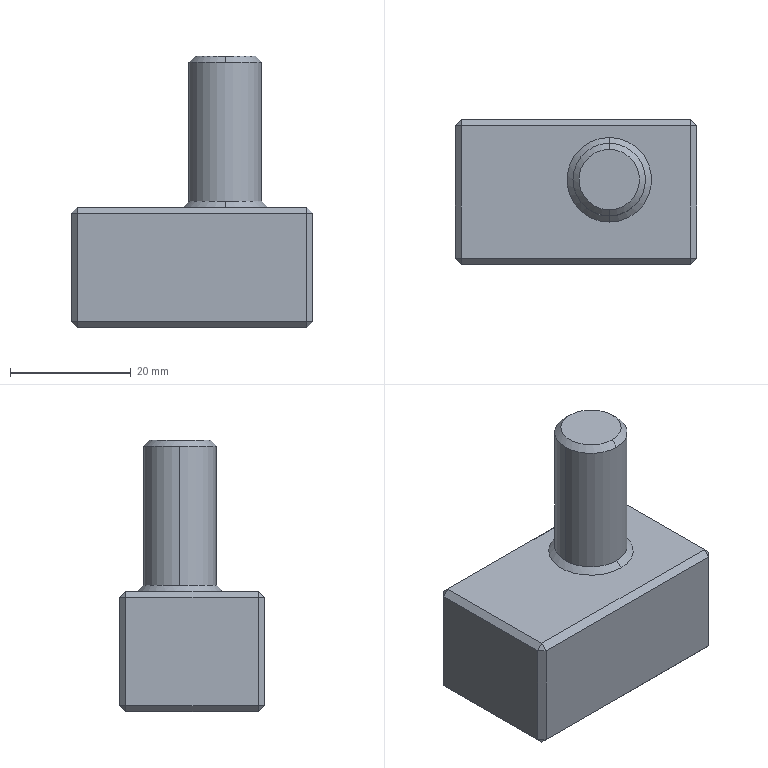Component | SolidWorks | LocatingPinB-1 | 1 solid | 33 faces | box 40 x 24 x 45 mm | volume 21867 mm3 | plane 27 | cone 4 | cylinder 2 | commonest cylinder face diameters 12 x2 | material Aviation Aluminum-7075
build123d program:
from build123d import *

# Parameters (mm, degrees)
SKETCH1_W           = 40
SKETCH1_H           = 20
BOSS_EXTRUDE1_DEPTH = 24
SKETCH2_R           = 6
BOSS_EXTRUDE2_DEPTH = 25
CHAMFER1_SIZE       = 1


with BuildPart() as part:
    # Sketch1 → Boss-Extrude1 (new body)
    with BuildSketch(Plane.XY):
        Rectangle(SKETCH1_W, SKETCH1_H)
    extrude(amount=BOSS_EXTRUDE1_DEPTH)

    # Sketch2 → Boss-Extrude2 (add)
    with BuildSketch(Plane.XZ.offset(10)):
        with Locations(Location((5.5, 14, 0), (0, 0, 180))):
            Circle(SKETCH2_R)
    extrude(amount=BOSS_EXTRUDE2_DEPTH)

    # Chamfer1
    chamfer1_edges = [part.edges().sort_by_distance(p)[0] for p in [
        (20, 0, 24),
        (0, 10, 24),
        (11.5, -10, 14),
        (11.5, -35, 14),
        (-20, 0, 24),
        (0, 10, 0),
        (20, 0, 0),
        (0, -10, 0),
        (-20, 0, 0),
        (0, -10, 24),
        (-20, 10, 12),
        (20, 10, 12),
        (20, -10, 12),
        (-20, -10, 12),
    ]]
    chamfer(chamfer1_edges, length=CHAMFER1_SIZE)


solid = part.part

# Placed as in the assembly
solid = solid.moved(Location((85.13, -406.626, 682.215), (-90, 0, 0)))
STEP:
#1=CARTESIAN_POINT('',(3.568,-15.655,28.237));
#2=VERTEX_POINT('',#1);
#3=CARTESIAN_POINT('',(3.568,-15.261,28.237));
#4=VERTEX_POINT('',#3);
#5=CARTESIAN_POINT('',(3.568,-15.458,28.237));
#6=DIRECTION('',(0.,-0.,1.));
#7=DIRECTION('',(1.,0.,0.));
#8=AXIS2_PLACEMENT_3D('',#5,#6,#7);
#9=CIRCLE('',#8,0.1969);
#10=EDGE_CURVE('',#2,#4,#9,.T.);
#11=ORIENTED_EDGE('',*,*,#10,.F.);
#12=CARTESIAN_POINT('',(3.568,-15.694,28.197));
#13=VERTEX_POINT('',#12);
#14=CARTESIAN_POINT('',(3.568,-15.655,28.237));
#15=DIRECTION('',(-0.,-0.7071,-0.7071));
#16=VECTOR('',#15,39.37);
#17=LINE('',#14,#16);
#18=EDGE_CURVE('',#2,#13,#17,.T.);
#19=ORIENTED_EDGE('',*,*,#18,.T.);
#20=CARTESIAN_POINT('',(3.804,-15.458,28.197));
#21=VERTEX_POINT('',#20);
#22=CARTESIAN_POINT('',(3.568,-15.458,28.197));
#23=DIRECTION('',(-0.,0.,-1.));
#24=DIRECTION('',(0.,-1.,0.));
#25=AXIS2_PLACEMENT_3D('',#22,#23,#24);
#26=CIRCLE('',#25,0.2362);
#27=EDGE_CURVE('',#21,#13,#26,.T.);
#28=ORIENTED_EDGE('',*,*,#27,.F.);
#29=CARTESIAN_POINT('',(3.568,-15.222,28.197));
#30=VERTEX_POINT('',#29);
#31=CARTESIAN_POINT('',(3.568,-15.458,28.197));
#32=DIRECTION('',(-0.,0.,-1.));
#33=DIRECTION('',(0.,-1.,0.));
#34=AXIS2_PLACEMENT_3D('',#31,#32,#33);
#35=CIRCLE('',#34,0.2362);
#36=EDGE_CURVE('',#30,#21,#35,.T.);
#37=ORIENTED_EDGE('',*,*,#36,.F.);
#38=CARTESIAN_POINT('',(3.568,-15.261,28.237));
#39=DIRECTION('',(-0.,0.7071,-0.7071));
#40=VECTOR('',#39,39.37);
#41=LINE('',#38,#40);
#42=EDGE_CURVE('',#4,#30,#41,.T.);
#43=ORIENTED_EDGE('',*,*,#42,.F.);
#44=EDGE_LOOP('',(#11,#19,#28,#37,#43));
#45=FACE_OUTER_BOUND('',#44,.T.);
#46=CARTESIAN_POINT('',(3.568,-15.458,28.237));
#47=DIRECTION('',(-0.,0.,-1.));
#48=DIRECTION('',(0.,1.,0.));
#49=AXIS2_PLACEMENT_3D('',#46,#47,#48);
#50=CONICAL_SURFACE('',#49,0.1969,0.7854);
#51=ADVANCED_FACE('',(#45),#50,.T.);
#52=CARTESIAN_POINT('',(3.568,-15.694,27.292));
#53=VERTEX_POINT('',#52);
#54=CARTESIAN_POINT('',(3.804,-15.458,27.292));
#55=VERTEX_POINT('',#54);
#56=CARTESIAN_POINT('',(3.568,-15.458,27.292));
#57=DIRECTION('',(0.,-0.,1.));
#58=DIRECTION('',(0.,1.,0.));
#59=AXIS2_PLACEMENT_3D('',#56,#57,#58);
#60=CIRCLE('',#59,0.2362);
#61=EDGE_CURVE('',#53,#55,#60,.T.);
#62=ORIENTED_EDGE('',*,*,#61,.F.);
#63=CARTESIAN_POINT('',(3.568,-15.733,27.253));
#64=VERTEX_POINT('',#63);
#65=CARTESIAN_POINT('',(3.568,-15.694,27.292));
#66=DIRECTION('',(-0.,-0.7071,-0.7071));
#67=VECTOR('',#66,39.37);
#68=LINE('',#65,#67);
#69=EDGE_CURVE('',#53,#64,#68,.T.);
#70=ORIENTED_EDGE('',*,*,#69,.T.);
#71=CARTESIAN_POINT('',(3.568,-15.182,27.253));
#72=VERTEX_POINT('',#71);
#73=CARTESIAN_POINT('',(3.568,-15.458,27.253));
#74=DIRECTION('',(-0.,0.,-1.));
#75=DIRECTION('',(-1.,0.,0.));
#76=AXIS2_PLACEMENT_3D('',#73,#74,#75);
#77=CIRCLE('',#76,0.2756);
#78=EDGE_CURVE('',#72,#64,#77,.T.);
#79=ORIENTED_EDGE('',*,*,#78,.F.);
#80=CARTESIAN_POINT('',(3.568,-15.222,27.292));
#81=VERTEX_POINT('',#80);
#82=CARTESIAN_POINT('',(3.568,-15.222,27.292));
#83=DIRECTION('',(-0.,0.7071,-0.7071));
#84=VECTOR('',#83,39.37);
#85=LINE('',#82,#84);
#86=EDGE_CURVE('',#81,#72,#85,.T.);
#87=ORIENTED_EDGE('',*,*,#86,.F.);
#88=CARTESIAN_POINT('',(3.568,-15.458,27.292));
#89=DIRECTION('',(0.,-0.,1.));
#90=DIRECTION('',(0.,1.,0.));
#91=AXIS2_PLACEMENT_3D('',#88,#89,#90);
#92=CIRCLE('',#91,0.2362);
#93=EDGE_CURVE('',#55,#81,#92,.T.);
#94=ORIENTED_EDGE('',*,*,#93,.F.);
#95=EDGE_LOOP('',(#62,#70,#79,#87,#94));
#96=FACE_OUTER_BOUND('',#95,.T.);
#97=CARTESIAN_POINT('',(3.568,-15.458,27.292));
#98=DIRECTION('',(-0.,0.,-1.));
#99=DIRECTION('',(0.,1.,0.));
#100=AXIS2_PLACEMENT_3D('',#97,#98,#99);
#101=CONICAL_SURFACE('',#100,0.2362,0.7854);
#102=ADVANCED_FACE('',(#96),#101,.T.);
#103=CARTESIAN_POINT('',(3.332,-15.458,28.197));
#104=VERTEX_POINT('',#103);
#105=CARTESIAN_POINT('',(3.568,-15.458,28.197));
#106=DIRECTION('',(-0.,0.,-1.));
#107=DIRECTION('',(0.,-1.,0.));
#108=AXIS2_PLACEMENT_3D('',#105,#106,#107);
#109=CIRCLE('',#108,0.2362);
#110=EDGE_CURVE('',#104,#30,#109,.T.);
#111=ORIENTED_EDGE('',*,*,#110,.T.);
#112=ORIENTED_EDGE('',*,*,#36,.T.);
#113=CARTESIAN_POINT('',(3.804,-15.458,28.237));
#114=DIRECTION('',(-0.,0.,-1.));
#115=VECTOR('',#114,39.37);
#116=LINE('',#113,#115);
#117=EDGE_CURVE('',#21,#55,#116,.T.);
#118=ORIENTED_EDGE('',*,*,#117,.T.);
#119=ORIENTED_EDGE('',*,*,#93,.T.);
#120=CARTESIAN_POINT('',(3.332,-15.458,27.292));
#121=VERTEX_POINT('',#120);
#122=CARTESIAN_POINT('',(3.568,-15.458,27.292));
#123=DIRECTION('',(0.,-0.,1.));
#124=DIRECTION('',(0.,1.,0.));
#125=AXIS2_PLACEMENT_3D('',#122,#123,#124);
#126=CIRCLE('',#125,0.2362);
#127=EDGE_CURVE('',#81,#121,#126,.T.);
#128=ORIENTED_EDGE('',*,*,#127,.T.);
#129=CARTESIAN_POINT('',(3.332,-15.458,28.237));
#130=DIRECTION('',(-0.,0.,-1.));
#131=VECTOR('',#130,39.37);
#132=LINE('',#129,#131);
#133=EDGE_CURVE('',#104,#121,#132,.T.);
#134=ORIENTED_EDGE('',*,*,#133,.F.);
#135=EDGE_LOOP('',(#111,#112,#118,#119,#128,#134));
#136=FACE_OUTER_BOUND('',#135,.T.);
#137=CARTESIAN_POINT('',(3.568,-15.458,28.237));
#138=DIRECTION('',(-0.,0.,-1.));
#139=DIRECTION('',(-1.,0.,0.));
#140=AXIS2_PLACEMENT_3D('',#137,#138,#139);
#141=CYLINDRICAL_SURFACE('',#140,0.2362);
#142=ADVANCED_FACE('',(#136),#141,.T.);
#143=ORIENTED_EDGE('',*,*,#78,.T.);
#144=CARTESIAN_POINT('',(3.568,-15.458,27.253));
#145=DIRECTION('',(-0.,0.,-1.));
#146=DIRECTION('',(-1.,0.,0.));
#147=AXIS2_PLACEMENT_3D('',#144,#145,#146);
#148=CIRCLE('',#147,0.2756);
#149=EDGE_CURVE('',#64,#72,#148,.T.);
#150=ORIENTED_EDGE('',*,*,#149,.T.);
#151=EDGE_LOOP('',(#143,#150));
#152=FACE_BOUND('',#151,.T.);
#153=CARTESIAN_POINT('',(2.604,-15.97,27.253));
#154=VERTEX_POINT('',#153);
#155=CARTESIAN_POINT('',(4.1,-15.97,27.253));
#156=VERTEX_POINT('',#155);
#157=CARTESIAN_POINT('',(4.139,-15.97,27.253));
#158=DIRECTION('',(1.,-0.,-0.));
#159=VECTOR('',#158,39.37);
#160=LINE('',#157,#159);
#161=EDGE_CURVE('',#154,#156,#160,.T.);
#162=ORIENTED_EDGE('',*,*,#161,.T.);
#163=CARTESIAN_POINT('',(4.1,-15.103,27.253));
#164=VERTEX_POINT('',#163);
#165=CARTESIAN_POINT('',(4.1,-15.064,27.253));
#166=DIRECTION('',(0.,1.,0.));
#167=VECTOR('',#166,39.37);
#168=LINE('',#165,#167);
#169=EDGE_CURVE('',#156,#164,#168,.T.);
#170=ORIENTED_EDGE('',*,*,#169,.T.);
#171=CARTESIAN_POINT('',(2.604,-15.103,27.253));
#172=VERTEX_POINT('',#171);
#173=CARTESIAN_POINT('',(2.564,-15.103,27.253));
#174=DIRECTION('',(-1.,0.,0.));
#175=VECTOR('',#174,39.37);
#176=LINE('',#173,#175);
#177=EDGE_CURVE('',#164,#172,#176,.T.);
#178=ORIENTED_EDGE('',*,*,#177,.T.);
#179=CARTESIAN_POINT('',(2.604,-15.064,27.253));
#180=DIRECTION('',(-0.,-1.,-0.));
#181=VECTOR('',#180,39.37);
#182=LINE('',#179,#181);
#183=EDGE_CURVE('',#172,#154,#182,.T.);
#184=ORIENTED_EDGE('',*,*,#183,.T.);
#185=EDGE_LOOP('',(#162,#170,#178,#184));
#186=FACE_OUTER_BOUND('',#185,.T.);
#187=CARTESIAN_POINT('',(4.139,-15.064,27.253));
#188=DIRECTION('',(-0.,0.,-1.));
#189=DIRECTION('',(-1.,0.,0.));
#190=AXIS2_PLACEMENT_3D('',#187,#188,#189);
#191=PLANE('',#190);
#192=ADVANCED_FACE('',(#152,#186),#191,.F.);
#193=CARTESIAN_POINT('',(2.564,-15.97,26.505));
#194=VERTEX_POINT('',#193);
#195=CARTESIAN_POINT('',(2.564,-15.97,27.213));
#196=VERTEX_POINT('',#195);
#197=CARTESIAN_POINT('',(2.564,-15.97,27.253));
#198=DIRECTION('',(0.,-0.,1.));
#199=VECTOR('',#198,39.37);
#200=LINE('',#197,#199);
#201=EDGE_CURVE('',#194,#196,#200,.T.);
#202=ORIENTED_EDGE('',*,*,#201,.T.);
#203=CARTESIAN_POINT('',(2.564,-15.103,27.213));
#204=VERTEX_POINT('',#203);
#205=CARTESIAN_POINT('',(2.564,-15.064,27.213));
#206=DIRECTION('',(0.,1.,0.));
#207=VECTOR('',#206,39.37);
#208=LINE('',#205,#207);
#209=EDGE_CURVE('',#196,#204,#208,.T.);
#210=ORIENTED_EDGE('',*,*,#209,.T.);
#211=CARTESIAN_POINT('',(2.564,-15.103,26.505));
#212=VERTEX_POINT('',#211);
#213=CARTESIAN_POINT('',(2.564,-15.103,26.465));
#214=DIRECTION('',(-0.,0.,-1.));
#215=VECTOR('',#214,39.37);
#216=LINE('',#213,#215);
#217=EDGE_CURVE('',#204,#212,#216,.T.);
#218=ORIENTED_EDGE('',*,*,#217,.T.);
#219=CARTESIAN_POINT('',(2.564,-15.064,26.505));
#220=DIRECTION('',(-0.,-1.,-0.));
#221=VECTOR('',#220,39.37);
#222=LINE('',#219,#221);
#223=EDGE_CURVE('',#212,#194,#222,.T.);
#224=ORIENTED_EDGE('',*,*,#223,.T.);
#225=EDGE_LOOP('',(#202,#210,#218,#224));
#226=FACE_OUTER_BOUND('',#225,.T.);
#227=CARTESIAN_POINT('',(2.564,-15.064,27.253));
#228=DIRECTION('',(1.,-0.,-0.));
#229=DIRECTION('',(-0.,0.,-1.));
#230=AXIS2_PLACEMENT_3D('',#227,#228,#229);
#231=PLANE('',#230);
#232=ADVANCED_FACE('',(#226),#231,.F.);
#233=CARTESIAN_POINT('',(4.139,-15.103,26.505));
#234=VERTEX_POINT('',#233);
#235=CARTESIAN_POINT('',(4.139,-15.103,27.213));
#236=VERTEX_POINT('',#235);
#237=CARTESIAN_POINT('',(4.139,-15.103,27.253));
#238=DIRECTION('',(0.,-0.,1.));
#239=VECTOR('',#238,39.37);
#240=LINE('',#237,#239);
#241=EDGE_CURVE('',#234,#236,#240,.T.);
#242=ORIENTED_EDGE('',*,*,#241,.T.);
#243=CARTESIAN_POINT('',(4.139,-15.97,27.213));
#244=VERTEX_POINT('',#243);
#245=CARTESIAN_POINT('',(4.139,-15.064,27.213));
#246=DIRECTION('',(-0.,-1.,-0.));
#247=VECTOR('',#246,39.37);
#248=LINE('',#245,#247);
#249=EDGE_CURVE('',#236,#244,#248,.T.);
#250=ORIENTED_EDGE('',*,*,#249,.T.);
#251=CARTESIAN_POINT('',(4.139,-15.97,26.505));
#252=VERTEX_POINT('',#251);
#253=CARTESIAN_POINT('',(4.139,-15.97,27.253));
#254=DIRECTION('',(-0.,0.,-1.));
#255=VECTOR('',#254,39.37);
#256=LINE('',#253,#255);
#257=EDGE_CURVE('',#244,#252,#256,.T.);
#258=ORIENTED_EDGE('',*,*,#257,.T.);
#259=CARTESIAN_POINT('',(4.139,-15.064,26.505));
#260=DIRECTION('',(0.,1.,0.));
#261=VECTOR('',#260,39.37);
#262=LINE('',#259,#261);
#263=EDGE_CURVE('',#252,#234,#262,.T.);
#264=ORIENTED_EDGE('',*,*,#263,.T.);
#265=EDGE_LOOP('',(#242,#250,#258,#264));
#266=FACE_OUTER_BOUND('',#265,.T.);
#267=CARTESIAN_POINT('',(4.139,-15.064,27.253));
#268=DIRECTION('',(-1.,0.,0.));
#269=DIRECTION('',(0.,1.,0.));
#270=AXIS2_PLACEMENT_3D('',#267,#268,#269);
#271=PLANE('',#270);
#272=ADVANCED_FACE('',(#266),#271,.F.);
#273=CARTESIAN_POINT('',(2.604,-15.103,26.465));
#274=VERTEX_POINT('',#273);
#275=CARTESIAN_POINT('',(4.1,-15.103,26.465));
#276=VERTEX_POINT('',#275);
#277=CARTESIAN_POINT('',(4.139,-15.103,26.465));
#278=DIRECTION('',(1.,-0.,-0.));
#279=VECTOR('',#278,39.37);
#280=LINE('',#277,#279);
#281=EDGE_CURVE('',#274,#276,#280,.T.);
#282=ORIENTED_EDGE('',*,*,#281,.T.);
#283=CARTESIAN_POINT('',(4.1,-15.97,26.465));
#284=VERTEX_POINT('',#283);
#285=CARTESIAN_POINT('',(4.1,-15.064,26.465));
#286=DIRECTION('',(-0.,-1.,-0.));
#287=VECTOR('',#286,39.37);
#288=LINE('',#285,#287);
#289=EDGE_CURVE('',#276,#284,#288,.T.);
#290=ORIENTED_EDGE('',*,*,#289,.T.);
#291=CARTESIAN_POINT('',(2.604,-15.97,26.465));
#292=VERTEX_POINT('',#291);
#293=CARTESIAN_POINT('',(4.139,-15.97,26.465));
#294=DIRECTION('',(-1.,0.,0.));
#295=VECTOR('',#294,39.37);
#296=LINE('',#293,#295);
#297=EDGE_CURVE('',#284,#292,#296,.T.);
#298=ORIENTED_EDGE('',*,*,#297,.T.);
#299=CARTESIAN_POINT('',(2.604,-15.064,26.465));
#300=DIRECTION('',(0.,1.,0.));
#301=VECTOR('',#300,39.37);
#302=LINE('',#299,#301);
#303=EDGE_CURVE('',#292,#274,#302,.T.);
#304=ORIENTED_EDGE('',*,*,#303,.T.);
#305=EDGE_LOOP('',(#282,#290,#298,#304));
#306=FACE_OUTER_BOUND('',#305,.T.);
#307=CARTESIAN_POINT('',(4.139,-15.064,26.465));
#308=DIRECTION('',(0.,-0.,1.));
#309=DIRECTION('',(1.,-0.,-0.));
#310=AXIS2_PLACEMENT_3D('',#307,#308,#309);
#311=PLANE('',#310);
#312=ADVANCED_FACE('',(#306),#311,.F.);
#313=CARTESIAN_POINT('',(2.604,-15.064,27.213));
#314=VERTEX_POINT('',#313);
#315=CARTESIAN_POINT('',(4.1,-15.064,27.213));
#316=VERTEX_POINT('',#315);
#317=CARTESIAN_POINT('',(4.139,-15.064,27.213));
#318=DIRECTION('',(1.,-0.,-0.));
#319=VECTOR('',#318,39.37);
#320=LINE('',#317,#319);
#321=EDGE_CURVE('',#314,#316,#320,.T.);
#322=ORIENTED_EDGE('',*,*,#321,.T.);
#323=CARTESIAN_POINT('',(4.1,-15.064,26.505));
#324=VERTEX_POINT('',#323);
#325=CARTESIAN_POINT('',(4.1,-15.064,26.465));
#326=DIRECTION('',(-0.,0.,-1.));
#327=VECTOR('',#326,39.37);
#328=LINE('',#325,#327);
#329=EDGE_CURVE('',#316,#324,#328,.T.);
#330=ORIENTED_EDGE('',*,*,#329,.T.);
#331=CARTESIAN_POINT('',(2.604,-15.064,26.505));
#332=VERTEX_POINT('',#331);
#333=CARTESIAN_POINT('',(2.564,-15.064,26.505));
#334=DIRECTION('',(-1.,0.,0.));
#335=VECTOR('',#334,39.37);
#336=LINE('',#333,#335);
#337=EDGE_CURVE('',#324,#332,#336,.T.);
#338=ORIENTED_EDGE('',*,*,#337,.T.);
#339=CARTESIAN_POINT('',(2.604,-15.064,27.253));
#340=DIRECTION('',(0.,-0.,1.));
#341=VECTOR('',#340,39.37);
#342=LINE('',#339,#341);
#343=EDGE_CURVE('',#332,#314,#342,.T.);
#344=ORIENTED_EDGE('',*,*,#343,.T.);
#345=EDGE_LOOP('',(#322,#330,#338,#344));
#346=FACE_OUTER_BOUND('',#345,.T.);
#347=CARTESIAN_POINT('',(3.352,-15.064,26.859));
#348=DIRECTION('',(0.,1.,0.));
#349=DIRECTION('',(1.,-0.,-0.));
#350=AXIS2_PLACEMENT_3D('',#347,#348,#349);
#351=PLANE('',#350);
#352=ADVANCED_FACE('',(#346),#351,.T.);
#353=CARTESIAN_POINT('',(4.1,-16.009,26.505));
#354=VERTEX_POINT('',#353);
#355=CARTESIAN_POINT('',(4.1,-16.009,27.213));
#356=VERTEX_POINT('',#355);
#357=CARTESIAN_POINT('',(4.1,-16.009,26.859));
#358=DIRECTION('',(0.,-0.,1.));
#359=VECTOR('',#358,39.37);
#360=LINE('',#357,#359);
#361=EDGE_CURVE('',#354,#356,#360,.T.);
#362=ORIENTED_EDGE('',*,*,#361,.T.);
#363=CARTESIAN_POINT('',(2.604,-16.009,27.213));
#364=VERTEX_POINT('',#363);
#365=CARTESIAN_POINT('',(3.352,-16.009,27.213));
#366=DIRECTION('',(-1.,0.,0.));
#367=VECTOR('',#366,39.37);
#368=LINE('',#365,#367);
#369=EDGE_CURVE('',#356,#364,#368,.T.);
#370=ORIENTED_EDGE('',*,*,#369,.T.);
#371=CARTESIAN_POINT('',(2.604,-16.009,26.505));
#372=VERTEX_POINT('',#371);
#373=CARTESIAN_POINT('',(2.604,-16.009,26.859));
#374=DIRECTION('',(-0.,0.,-1.));
#375=VECTOR('',#374,39.37);
#376=LINE('',#373,#375);
#377=EDGE_CURVE('',#364,#372,#376,.T.);
#378=ORIENTED_EDGE('',*,*,#377,.T.);
#379=CARTESIAN_POINT('',(3.352,-16.009,26.505));
#380=DIRECTION('',(1.,-0.,-0.));
#381=VECTOR('',#380,39.37);
#382=LINE('',#379,#381);
#383=EDGE_CURVE('',#372,#354,#382,.T.);
#384=ORIENTED_EDGE('',*,*,#383,.T.);
#385=EDGE_LOOP('',(#362,#370,#378,#384));
#386=FACE_OUTER_BOUND('',#385,.T.);
#387=CARTESIAN_POINT('',(3.352,-16.009,26.859));
#388=DIRECTION('',(0.,1.,0.));
#389=DIRECTION('',(1.,-0.,-0.));
#390=AXIS2_PLACEMENT_3D('',#387,#388,#389);
#391=PLANE('',#390);
#392=ADVANCED_FACE('',(#386),#391,.F.);
#393=ORIENTED_EDGE('',*,*,#117,.F.);
#394=ORIENTED_EDGE('',*,*,#27,.T.);
#395=CARTESIAN_POINT('',(3.568,-15.458,28.197));
#396=DIRECTION('',(-0.,0.,-1.));
#397=DIRECTION('',(0.,-1.,0.));
#398=AXIS2_PLACEMENT_3D('',#395,#396,#397);
#399=CIRCLE('',#398,0.2362);
#400=EDGE_CURVE('',#13,#104,#399,.T.);
#401=ORIENTED_EDGE('',*,*,#400,.T.);
#402=ORIENTED_EDGE('',*,*,#133,.T.);
#403=CARTESIAN_POINT('',(3.568,-15.458,27.292));
#404=DIRECTION('',(0.,-0.,1.));
#405=DIRECTION('',(0.,1.,0.));
#406=AXIS2_PLACEMENT_3D('',#403,#404,#405);
#407=CIRCLE('',#406,0.2362);
#408=EDGE_CURVE('',#121,#53,#407,.T.);
#409=ORIENTED_EDGE('',*,*,#408,.T.);
#410=ORIENTED_EDGE('',*,*,#61,.T.);
#411=EDGE_LOOP('',(#393,#394,#401,#402,#409,#410));
#412=FACE_OUTER_BOUND('',#411,.T.);
#413=CARTESIAN_POINT('',(3.568,-15.458,28.237));
#414=DIRECTION('',(-0.,0.,-1.));
#415=DIRECTION('',(-1.,0.,0.));
#416=AXIS2_PLACEMENT_3D('',#413,#414,#415);
#417=CYLINDRICAL_SURFACE('',#416,0.2362);
#418=ADVANCED_FACE('',(#412),#417,.T.);
#419=CARTESIAN_POINT('',(3.568,-15.458,28.237));
#420=DIRECTION('',(0.,-0.,1.));
#421=DIRECTION('',(1.,0.,0.));
#422=AXIS2_PLACEMENT_3D('',#419,#420,#421);
#423=CIRCLE('',#422,0.1969);
#424=EDGE_CURVE('',#4,#2,#423,.T.);
#425=ORIENTED_EDGE('',*,*,#424,.T.);
#426=ORIENTED_EDGE('',*,*,#10,.T.);
#427=EDGE_LOOP('',(#425,#426));
#428=FACE_OUTER_BOUND('',#427,.T.);
#429=CARTESIAN_POINT('',(3.568,-15.458,28.237));
#430=DIRECTION('',(0.,-0.,1.));
#431=DIRECTION('',(1.,-0.,-0.));
#432=AXIS2_PLACEMENT_3D('',#429,#430,#431);
#433=PLANE('',#432);
#434=ADVANCED_FACE('',(#428),#433,.T.);
#435=ORIENTED_EDGE('',*,*,#69,.F.);
#436=ORIENTED_EDGE('',*,*,#408,.F.);
#437=ORIENTED_EDGE('',*,*,#127,.F.);
#438=ORIENTED_EDGE('',*,*,#86,.T.);
#439=ORIENTED_EDGE('',*,*,#149,.F.);
#440=EDGE_LOOP('',(#435,#436,#437,#438,#439));
#441=FACE_OUTER_BOUND('',#440,.T.);
#442=CARTESIAN_POINT('',(3.568,-15.458,27.292));
#443=DIRECTION('',(-0.,0.,-1.));
#444=DIRECTION('',(0.,1.,0.));
#445=AXIS2_PLACEMENT_3D('',#442,#443,#444);
#446=CONICAL_SURFACE('',#445,0.2362,0.7854);
#447=ADVANCED_FACE('',(#441),#446,.T.);
#448=CARTESIAN_POINT('',(2.564,-15.103,26.505));
#449=DIRECTION('',(-0.7071,-0.,0.7071));
#450=VECTOR('',#449,39.37);
#451=LINE('',#448,#450);
#452=EDGE_CURVE('',#274,#212,#451,.T.);
#453=ORIENTED_EDGE('',*,*,#452,.F.);
#454=ORIENTED_EDGE('',*,*,#303,.F.);
#455=CARTESIAN_POINT('',(2.584,-15.97,26.485));
#456=DIRECTION('',(0.7071,-0.,-0.7071));
#457=VECTOR('',#456,39.37);
#458=LINE('',#455,#457);
#459=EDGE_CURVE('',#194,#292,#458,.T.);
#460=ORIENTED_EDGE('',*,*,#459,.F.);
#461=ORIENTED_EDGE('',*,*,#223,.F.);
#462=EDGE_LOOP('',(#453,#454,#460,#461));
#463=FACE_OUTER_BOUND('',#462,.T.);
#464=CARTESIAN_POINT('',(2.564,-15.064,26.505));
#465=DIRECTION('',(0.7071,-0.,0.7071));
#466=DIRECTION('',(-0.,-1.,-0.));
#467=AXIS2_PLACEMENT_3D('',#464,#465,#466);
#468=PLANE('',#467);
#469=ADVANCED_FACE('',(#463),#468,.F.);
#470=CARTESIAN_POINT('',(2.604,-15.084,26.485));
#471=DIRECTION('',(-0.,0.7071,0.7071));
#472=VECTOR('',#471,39.37);
#473=LINE('',#470,#472);
#474=EDGE_CURVE('',#274,#332,#473,.T.);
#475=ORIENTED_EDGE('',*,*,#474,.F.);
#476=ORIENTED_EDGE('',*,*,#452,.T.);
#477=CARTESIAN_POINT('',(2.564,-15.103,26.505));
#478=DIRECTION('',(-0.7071,-0.7071,0.));
#479=VECTOR('',#478,39.37);
#480=LINE('',#477,#479);
#481=EDGE_CURVE('',#332,#212,#480,.T.);
#482=ORIENTED_EDGE('',*,*,#481,.F.);
#483=EDGE_LOOP('',(#475,#476,#482));
#484=FACE_OUTER_BOUND('',#483,.T.);
#485=CARTESIAN_POINT('',(2.564,-15.103,26.505));
#486=DIRECTION('',(-0.5774,0.5774,-0.5774));
#487=DIRECTION('',(0.7071,0.7071,0.));
#488=AXIS2_PLACEMENT_3D('',#485,#486,#487);
#489=PLANE('',#488);
#490=ADVANCED_FACE('',(#484),#489,.T.);
#491=CARTESIAN_POINT('',(2.604,-16.009,26.505));
#492=DIRECTION('',(0.7071,-0.7071,0.));
#493=VECTOR('',#492,39.37);
#494=LINE('',#491,#493);
#495=EDGE_CURVE('',#194,#372,#494,.T.);
#496=ORIENTED_EDGE('',*,*,#495,.F.);
#497=ORIENTED_EDGE('',*,*,#459,.T.);
#498=CARTESIAN_POINT('',(2.604,-16.009,26.505));
#499=DIRECTION('',(-0.,0.7071,-0.7071));
#500=VECTOR('',#499,39.37);
#501=LINE('',#498,#500);
#502=EDGE_CURVE('',#372,#292,#501,.T.);
#503=ORIENTED_EDGE('',*,*,#502,.F.);
#504=EDGE_LOOP('',(#496,#497,#503));
#505=FACE_OUTER_BOUND('',#504,.T.);
#506=CARTESIAN_POINT('',(2.604,-16.009,26.505));
#507=DIRECTION('',(-0.5774,-0.5774,-0.5774));
#508=DIRECTION('',(-0.7071,0.7071,0.));
#509=AXIS2_PLACEMENT_3D('',#506,#507,#508);
#510=PLANE('',#509);
#511=ADVANCED_FACE('',(#505),#510,.T.);
#512=ORIENTED_EDGE('',*,*,#481,.T.);
#513=ORIENTED_EDGE('',*,*,#217,.F.);
#514=CARTESIAN_POINT('',(2.564,-15.103,27.213));
#515=DIRECTION('',(-0.7071,-0.7071,-0.));
#516=VECTOR('',#515,39.37);
#517=LINE('',#514,#516);
#518=EDGE_CURVE('',#314,#204,#517,.T.);
#519=ORIENTED_EDGE('',*,*,#518,.F.);
#520=ORIENTED_EDGE('',*,*,#343,.F.);
#521=EDGE_LOOP('',(#512,#513,#519,#520));
#522=FACE_OUTER_BOUND('',#521,.T.);
#523=CARTESIAN_POINT('',(2.604,-15.064,26.859));
#524=DIRECTION('',(-0.7071,0.7071,0.));
#525=DIRECTION('',(-0.,0.,-1.));
#526=AXIS2_PLACEMENT_3D('',#523,#524,#525);
#527=PLANE('',#526);
#528=ADVANCED_FACE('',(#522),#527,.T.);
#529=ORIENTED_EDGE('',*,*,#474,.T.);
#530=ORIENTED_EDGE('',*,*,#337,.F.);
#531=CARTESIAN_POINT('',(4.1,-15.064,26.505));
#532=DIRECTION('',(0.,0.7071,0.7071));
#533=VECTOR('',#532,39.37);
#534=LINE('',#531,#533);
#535=EDGE_CURVE('',#276,#324,#534,.T.);
#536=ORIENTED_EDGE('',*,*,#535,.F.);
#537=ORIENTED_EDGE('',*,*,#281,.F.);
#538=EDGE_LOOP('',(#529,#530,#536,#537));
#539=FACE_OUTER_BOUND('',#538,.T.);
#540=CARTESIAN_POINT('',(3.352,-15.064,26.505));
#541=DIRECTION('',(-0.,0.7071,-0.7071));
#542=DIRECTION('',(1.,-0.,-0.));
#543=AXIS2_PLACEMENT_3D('',#540,#541,#542);
#544=PLANE('',#543);
#545=ADVANCED_FACE('',(#539),#544,.T.);
#546=CARTESIAN_POINT('',(4.139,-15.97,26.505));
#547=DIRECTION('',(0.7071,-0.,0.7071));
#548=VECTOR('',#547,39.37);
#549=LINE('',#546,#548);
#550=EDGE_CURVE('',#284,#252,#549,.T.);
#551=ORIENTED_EDGE('',*,*,#550,.F.);
#552=ORIENTED_EDGE('',*,*,#289,.F.);
#553=CARTESIAN_POINT('',(4.119,-15.103,26.485));
#554=DIRECTION('',(-0.7071,0.,-0.7071));
#555=VECTOR('',#554,39.37);
#556=LINE('',#553,#555);
#557=EDGE_CURVE('',#234,#276,#556,.T.);
#558=ORIENTED_EDGE('',*,*,#557,.F.);
#559=ORIENTED_EDGE('',*,*,#263,.F.);
#560=EDGE_LOOP('',(#551,#552,#558,#559));
#561=FACE_OUTER_BOUND('',#560,.T.);
#562=CARTESIAN_POINT('',(4.1,-15.064,26.465));
#563=DIRECTION('',(-0.7071,-0.,0.7071));
#564=DIRECTION('',(-0.,-1.,-0.));
#565=AXIS2_PLACEMENT_3D('',#562,#563,#564);
#566=PLANE('',#565);
#567=ADVANCED_FACE('',(#561),#566,.F.);
#568=ORIENTED_EDGE('',*,*,#502,.T.);
#569=ORIENTED_EDGE('',*,*,#297,.F.);
#570=CARTESIAN_POINT('',(4.1,-15.989,26.485));
#571=DIRECTION('',(0.,0.7071,-0.7071));
#572=VECTOR('',#571,39.37);
#573=LINE('',#570,#572);
#574=EDGE_CURVE('',#354,#284,#573,.T.);
#575=ORIENTED_EDGE('',*,*,#574,.F.);
#576=ORIENTED_EDGE('',*,*,#383,.F.);
#577=EDGE_LOOP('',(#568,#569,#575,#576));
#578=FACE_OUTER_BOUND('',#577,.T.);
#579=CARTESIAN_POINT('',(4.139,-15.97,26.465));
#580=DIRECTION('',(0.,0.7071,0.7071));
#581=DIRECTION('',(-1.,0.,0.));
#582=AXIS2_PLACEMENT_3D('',#579,#580,#581);
#583=PLANE('',#582);
#584=ADVANCED_FACE('',(#578),#583,.F.);
#585=ORIENTED_EDGE('',*,*,#495,.T.);
#586=ORIENTED_EDGE('',*,*,#377,.F.);
#587=CARTESIAN_POINT('',(2.604,-16.009,27.213));
#588=DIRECTION('',(0.7071,-0.7071,-0.));
#589=VECTOR('',#588,39.37);
#590=LINE('',#587,#589);
#591=EDGE_CURVE('',#196,#364,#590,.T.);
#592=ORIENTED_EDGE('',*,*,#591,.F.);
#593=ORIENTED_EDGE('',*,*,#201,.F.);
#594=EDGE_LOOP('',(#585,#586,#592,#593));
#595=FACE_OUTER_BOUND('',#594,.T.);
#596=CARTESIAN_POINT('',(2.564,-15.97,27.253));
#597=DIRECTION('',(0.7071,0.7071,0.));
#598=DIRECTION('',(0.,-0.,1.));
#599=AXIS2_PLACEMENT_3D('',#596,#597,#598);
#600=PLANE('',#599);
#601=ADVANCED_FACE('',(#595),#600,.F.);
#602=CARTESIAN_POINT('',(2.564,-15.103,27.213));
#603=DIRECTION('',(0.7071,-0.,0.7071));
#604=VECTOR('',#603,39.37);
#605=LINE('',#602,#604);
#606=EDGE_CURVE('',#204,#172,#605,.T.);
#607=ORIENTED_EDGE('',*,*,#606,.F.);
#608=ORIENTED_EDGE('',*,*,#209,.F.);
#609=CARTESIAN_POINT('',(2.584,-15.97,27.233));
#610=DIRECTION('',(-0.7071,0.,-0.7071));
#611=VECTOR('',#610,39.37);
#612=LINE('',#609,#611);
#613=EDGE_CURVE('',#154,#196,#612,.T.);
#614=ORIENTED_EDGE('',*,*,#613,.F.);
#615=ORIENTED_EDGE('',*,*,#183,.F.);
#616=EDGE_LOOP('',(#607,#608,#614,#615));
#617=FACE_OUTER_BOUND('',#616,.T.);
#618=CARTESIAN_POINT('',(2.604,-15.064,27.253));
#619=DIRECTION('',(0.7071,0.,-0.7071));
#620=DIRECTION('',(-0.,-1.,-0.));
#621=AXIS2_PLACEMENT_3D('',#618,#619,#620);
#622=PLANE('',#621);
#623=ADVANCED_FACE('',(#617),#622,.F.);
#624=ORIENTED_EDGE('',*,*,#518,.T.);
#625=ORIENTED_EDGE('',*,*,#606,.T.);
#626=CARTESIAN_POINT('',(2.604,-15.084,27.233));
#627=DIRECTION('',(-0.,-0.7071,0.7071));
#628=VECTOR('',#627,39.37);
#629=LINE('',#626,#628);
#630=EDGE_CURVE('',#314,#172,#629,.T.);
#631=ORIENTED_EDGE('',*,*,#630,.F.);
#632=EDGE_LOOP('',(#624,#625,#631));
#633=FACE_OUTER_BOUND('',#632,.T.);
#634=CARTESIAN_POINT('',(2.564,-15.103,27.213));
#635=DIRECTION('',(-0.5774,0.5774,0.5774));
#636=DIRECTION('',(0.7071,-0.,0.7071));
#637=AXIS2_PLACEMENT_3D('',#634,#635,#636);
#638=PLANE('',#637);
#639=ADVANCED_FACE('',(#633),#638,.T.);
#640=ORIENTED_EDGE('',*,*,#557,.T.);
#641=ORIENTED_EDGE('',*,*,#535,.T.);
#642=CARTESIAN_POINT('',(4.1,-15.064,26.505));
#643=DIRECTION('',(-0.7071,0.7071,0.));
#644=VECTOR('',#643,39.37);
#645=LINE('',#642,#644);
#646=EDGE_CURVE('',#234,#324,#645,.T.);
#647=ORIENTED_EDGE('',*,*,#646,.F.);
#648=EDGE_LOOP('',(#640,#641,#647));
#649=FACE_OUTER_BOUND('',#648,.T.);
#650=CARTESIAN_POINT('',(4.1,-15.064,26.505));
#651=DIRECTION('',(0.5774,0.5774,-0.5774));
#652=DIRECTION('',(0.7071,-0.7071,-0.));
#653=AXIS2_PLACEMENT_3D('',#650,#651,#652);
#654=PLANE('',#653);
#655=ADVANCED_FACE('',(#649),#654,.T.);
#656=ORIENTED_EDGE('',*,*,#574,.T.);
#657=ORIENTED_EDGE('',*,*,#550,.T.);
#658=CARTESIAN_POINT('',(4.139,-15.97,26.505));
#659=DIRECTION('',(0.7071,0.7071,-0.));
#660=VECTOR('',#659,39.37);
#661=LINE('',#658,#660);
#662=EDGE_CURVE('',#354,#252,#661,.T.);
#663=ORIENTED_EDGE('',*,*,#662,.F.);
#664=EDGE_LOOP('',(#656,#657,#663));
#665=FACE_OUTER_BOUND('',#664,.T.);
#666=CARTESIAN_POINT('',(4.139,-15.97,26.505));
#667=DIRECTION('',(0.5774,-0.5774,-0.5774));
#668=DIRECTION('',(-0.7071,-0.7071,-0.));
#669=AXIS2_PLACEMENT_3D('',#666,#667,#668);
#670=PLANE('',#669);
#671=ADVANCED_FACE('',(#665),#670,.T.);
#672=ORIENTED_EDGE('',*,*,#613,.T.);
#673=ORIENTED_EDGE('',*,*,#591,.T.);
#674=CARTESIAN_POINT('',(2.604,-16.009,27.213));
#675=DIRECTION('',(0.,-0.7071,-0.7071));
#676=VECTOR('',#675,39.37);
#677=LINE('',#674,#676);
#678=EDGE_CURVE('',#154,#364,#677,.T.);
#679=ORIENTED_EDGE('',*,*,#678,.F.);
#680=EDGE_LOOP('',(#672,#673,#679));
#681=FACE_OUTER_BOUND('',#680,.T.);
#682=CARTESIAN_POINT('',(2.604,-16.009,27.213));
#683=DIRECTION('',(-0.5774,-0.5774,0.5774));
#684=DIRECTION('',(-0.7071,0.7071,0.));
#685=AXIS2_PLACEMENT_3D('',#682,#683,#684);
#686=PLANE('',#685);
#687=ADVANCED_FACE('',(#681),#686,.T.);
#688=ORIENTED_EDGE('',*,*,#630,.T.);
#689=ORIENTED_EDGE('',*,*,#177,.F.);
#690=CARTESIAN_POINT('',(4.1,-15.103,27.253));
#691=DIRECTION('',(-0.,-0.7071,0.7071));
#692=VECTOR('',#691,39.37);
#693=LINE('',#690,#692);
#694=EDGE_CURVE('',#316,#164,#693,.T.);
#695=ORIENTED_EDGE('',*,*,#694,.F.);
#696=ORIENTED_EDGE('',*,*,#321,.F.);
#697=EDGE_LOOP('',(#688,#689,#695,#696));
#698=FACE_OUTER_BOUND('',#697,.T.);
#699=CARTESIAN_POINT('',(3.352,-15.064,27.213));
#700=DIRECTION('',(0.,0.7071,0.7071));
#701=DIRECTION('',(-1.,0.,0.));
#702=AXIS2_PLACEMENT_3D('',#699,#700,#701);
#703=PLANE('',#702);
#704=ADVANCED_FACE('',(#698),#703,.T.);
#705=ORIENTED_EDGE('',*,*,#646,.T.);
#706=ORIENTED_EDGE('',*,*,#329,.F.);
#707=CARTESIAN_POINT('',(4.119,-15.084,27.213));
#708=DIRECTION('',(-0.7071,0.7071,0.));
#709=VECTOR('',#708,39.37);
#710=LINE('',#707,#709);
#711=EDGE_CURVE('',#236,#316,#710,.T.);
#712=ORIENTED_EDGE('',*,*,#711,.F.);
#713=ORIENTED_EDGE('',*,*,#241,.F.);
#714=EDGE_LOOP('',(#705,#706,#712,#713));
#715=FACE_OUTER_BOUND('',#714,.T.);
#716=CARTESIAN_POINT('',(4.1,-15.064,26.859));
#717=DIRECTION('',(0.7071,0.7071,0.));
#718=DIRECTION('',(0.,-0.,1.));
#719=AXIS2_PLACEMENT_3D('',#716,#717,#718);
#720=PLANE('',#719);
#721=ADVANCED_FACE('',(#715),#720,.T.);
#722=ORIENTED_EDGE('',*,*,#662,.T.);
#723=ORIENTED_EDGE('',*,*,#257,.F.);
#724=CARTESIAN_POINT('',(4.139,-15.97,27.213));
#725=DIRECTION('',(0.7071,0.7071,0.));
#726=VECTOR('',#725,39.37);
#727=LINE('',#724,#726);
#728=EDGE_CURVE('',#356,#244,#727,.T.);
#729=ORIENTED_EDGE('',*,*,#728,.F.);
#730=ORIENTED_EDGE('',*,*,#361,.F.);
#731=EDGE_LOOP('',(#722,#723,#729,#730));
#732=FACE_OUTER_BOUND('',#731,.T.);
#733=CARTESIAN_POINT('',(4.139,-15.97,27.253));
#734=DIRECTION('',(-0.7071,0.7071,0.));
#735=DIRECTION('',(-0.,0.,-1.));
#736=AXIS2_PLACEMENT_3D('',#733,#734,#735);
#737=PLANE('',#736);
#738=ADVANCED_FACE('',(#732),#737,.F.);
#739=ORIENTED_EDGE('',*,*,#678,.T.);
#740=ORIENTED_EDGE('',*,*,#369,.F.);
#741=CARTESIAN_POINT('',(4.1,-15.989,27.233));
#742=DIRECTION('',(-0.,-0.7071,-0.7071));
#743=VECTOR('',#742,39.37);
#744=LINE('',#741,#743);
#745=EDGE_CURVE('',#156,#356,#744,.T.);
#746=ORIENTED_EDGE('',*,*,#745,.F.);
#747=ORIENTED_EDGE('',*,*,#161,.F.);
#748=EDGE_LOOP('',(#739,#740,#746,#747));
#749=FACE_OUTER_BOUND('',#748,.T.);
#750=CARTESIAN_POINT('',(4.139,-15.97,27.253));
#751=DIRECTION('',(-0.,0.7071,-0.7071));
#752=DIRECTION('',(1.,-0.,-0.));
#753=AXIS2_PLACEMENT_3D('',#750,#751,#752);
#754=PLANE('',#753);
#755=ADVANCED_FACE('',(#749),#754,.F.);
#756=ORIENTED_EDGE('',*,*,#711,.T.);
#757=ORIENTED_EDGE('',*,*,#694,.T.);
#758=CARTESIAN_POINT('',(4.1,-15.103,27.253));
#759=DIRECTION('',(-0.7071,-0.,0.7071));
#760=VECTOR('',#759,39.37);
#761=LINE('',#758,#760);
#762=EDGE_CURVE('',#236,#164,#761,.T.);
#763=ORIENTED_EDGE('',*,*,#762,.F.);
#764=EDGE_LOOP('',(#756,#757,#763));
#765=FACE_OUTER_BOUND('',#764,.T.);
#766=CARTESIAN_POINT('',(4.1,-15.103,27.253));
#767=DIRECTION('',(0.5774,0.5774,0.5774));
#768=DIRECTION('',(0.7071,0.,-0.7071));
#769=AXIS2_PLACEMENT_3D('',#766,#767,#768);
#770=PLANE('',#769);
#771=ADVANCED_FACE('',(#765),#770,.T.);
#772=ORIENTED_EDGE('',*,*,#745,.T.);
#773=ORIENTED_EDGE('',*,*,#728,.T.);
#774=CARTESIAN_POINT('',(4.139,-15.97,27.213));
#775=DIRECTION('',(0.7071,0.,-0.7071));
#776=VECTOR('',#775,39.37);
#777=LINE('',#774,#776);
#778=EDGE_CURVE('',#156,#244,#777,.T.);
#779=ORIENTED_EDGE('',*,*,#778,.F.);
#780=EDGE_LOOP('',(#772,#773,#779));
#781=FACE_OUTER_BOUND('',#780,.T.);
#782=CARTESIAN_POINT('',(4.139,-15.97,27.213));
#783=DIRECTION('',(0.5774,-0.5774,0.5774));
#784=DIRECTION('',(-0.,-0.7071,-0.7071));
#785=AXIS2_PLACEMENT_3D('',#782,#783,#784);
#786=PLANE('',#785);
#787=ADVANCED_FACE('',(#781),#786,.T.);
#788=ORIENTED_EDGE('',*,*,#762,.T.);
#789=ORIENTED_EDGE('',*,*,#169,.F.);
#790=ORIENTED_EDGE('',*,*,#778,.T.);
#791=ORIENTED_EDGE('',*,*,#249,.F.);
#792=EDGE_LOOP('',(#788,#789,#790,#791));
#793=FACE_OUTER_BOUND('',#792,.T.);
#794=CARTESIAN_POINT('',(4.139,-15.064,27.213));
#795=DIRECTION('',(-0.7071,0.,-0.7071));
#796=DIRECTION('',(-0.,-1.,-0.));
#797=AXIS2_PLACEMENT_3D('',#794,#795,#796);
#798=PLANE('',#797);
#799=ADVANCED_FACE('',(#793),#798,.F.);
#800=ORIENTED_EDGE('',*,*,#18,.F.);
#801=ORIENTED_EDGE('',*,*,#424,.F.);
#802=ORIENTED_EDGE('',*,*,#42,.T.);
#803=ORIENTED_EDGE('',*,*,#110,.F.);
#804=ORIENTED_EDGE('',*,*,#400,.F.);
#805=EDGE_LOOP('',(#800,#801,#802,#803,#804));
#806=FACE_OUTER_BOUND('',#805,.T.);
#807=CARTESIAN_POINT('',(3.568,-15.458,28.237));
#808=DIRECTION('',(-0.,0.,-1.));
#809=DIRECTION('',(0.,1.,0.));
#810=AXIS2_PLACEMENT_3D('',#807,#808,#809);
#811=CONICAL_SURFACE('',#810,0.1969,0.7854);
#812=ADVANCED_FACE('',(#806),#811,.T.);
#813=CLOSED_SHELL('',(#51,#102,#142,#192,#232,#272,#312,#352,#392,#418,#434,#447,#469,#490,#511,#528,#545,#567,#584,#601,#623,#639,#655,#671,#687,#704,#721,#738,#755,#771,#787,#799,#812));
#814=MANIFOLD_SOLID_BREP('',#813);
#815=CARTESIAN_POINT('',(0.,0.,0.));
#816=DIRECTION('',(0.,0.,1.));
#817=DIRECTION('',(1.,0.,0.));
#818=AXIS2_PLACEMENT_3D('',#815,#816,#817);
#819=(LENGTH_UNIT()NAMED_UNIT(*)SI_UNIT($,.METRE.));
#820=LENGTH_MEASURE_WITH_UNIT(LENGTH_MEASURE(0.0254),#819);
#821=DIMENSIONAL_EXPONENTS(1.,0.,0.,0.,0.,0.,0.);
#822=(CONVERSION_BASED_UNIT('',#820)LENGTH_UNIT()NAMED_UNIT(#821));
#823=UNCERTAINTY_MEASURE_WITH_UNIT(LENGTH_MEASURE(0.00001),#822,'','');
#824=(NAMED_UNIT(*)PLANE_ANGLE_UNIT()SI_UNIT($,.RADIAN.));
#825=(NAMED_UNIT(*)SI_UNIT($,.STERADIAN.)SOLID_ANGLE_UNIT());
#826=(GEOMETRIC_REPRESENTATION_CONTEXT(3)GLOBAL_UNCERTAINTY_ASSIGNED_CONTEXT((#823))GLOBAL_UNIT_ASSIGNED_CONTEXT((#822,#824,#825))REPRESENTATION_CONTEXT('',''));
#827=ADVANCED_BREP_SHAPE_REPRESENTATION('',(#814,#818),#826);
#828=COLOUR_RGB('',0.7922,0.8196,0.9333);
#829=FILL_AREA_STYLE_COLOUR('',#828);
#830=FILL_AREA_STYLE('',(#829));
#831=SURFACE_STYLE_FILL_AREA(#830);
#832=SURFACE_SIDE_STYLE('',(#831));
#833=SURFACE_STYLE_USAGE(.BOTH.,#832);
#834=PRESENTATION_STYLE_ASSIGNMENT((#833));
#835=STYLED_ITEM('',(#834),#814);
#836=(LENGTH_UNIT()NAMED_UNIT(*)SI_UNIT($,.METRE.));
#837=LENGTH_MEASURE_WITH_UNIT(LENGTH_MEASURE(0.0254),#836);
#838=DIMENSIONAL_EXPONENTS(1.,0.,0.,0.,0.,0.,0.);
#839=(CONVERSION_BASED_UNIT('',#837)LENGTH_UNIT()NAMED_UNIT(#838));
#840=UNCERTAINTY_MEASURE_WITH_UNIT(LENGTH_MEASURE(0.00001),#839,'','');
#841=(NAMED_UNIT(*)PLANE_ANGLE_UNIT()SI_UNIT($,.RADIAN.));
#842=(NAMED_UNIT(*)SI_UNIT($,.STERADIAN.)SOLID_ANGLE_UNIT());
#843=(GEOMETRIC_REPRESENTATION_CONTEXT(3)GLOBAL_UNCERTAINTY_ASSIGNED_CONTEXT((#840))GLOBAL_UNIT_ASSIGNED_CONTEXT((#839,#841,#842))REPRESENTATION_CONTEXT('',''));
#844=MECHANICAL_DESIGN_GEOMETRIC_PRESENTATION_REPRESENTATION('',(#835),#843);
#845=PRESENTATION_LAYER_ASSIGNMENT('','',(#835));